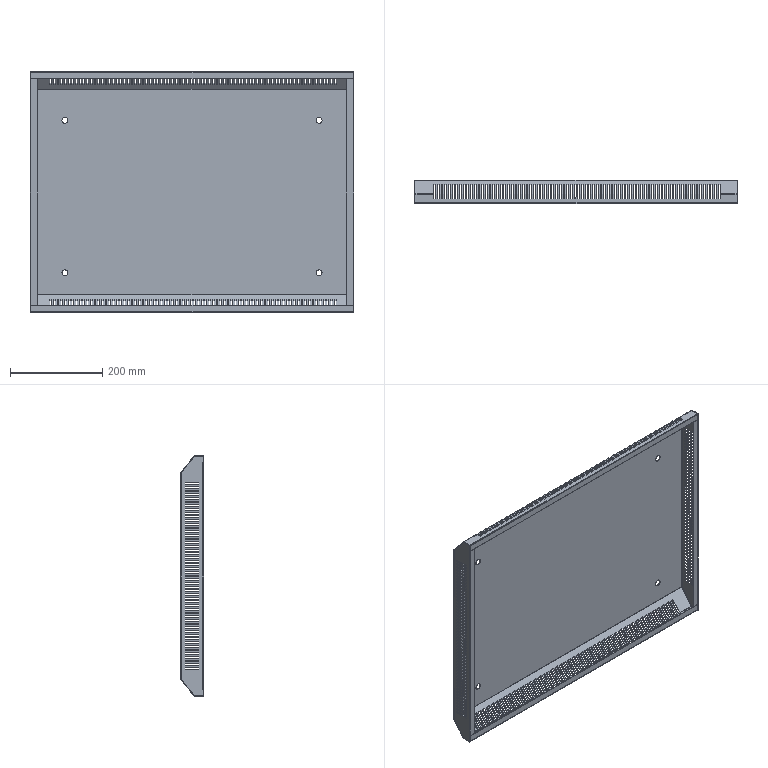Component | SolidWorks | KSHE-016.015-1 | 1 solid | 1474 faces | volume 535986 mm3 | plane 1134 | cylinder 340 | commonest cylinder face diameters 2.6 x166 0.2 x166 13 x8